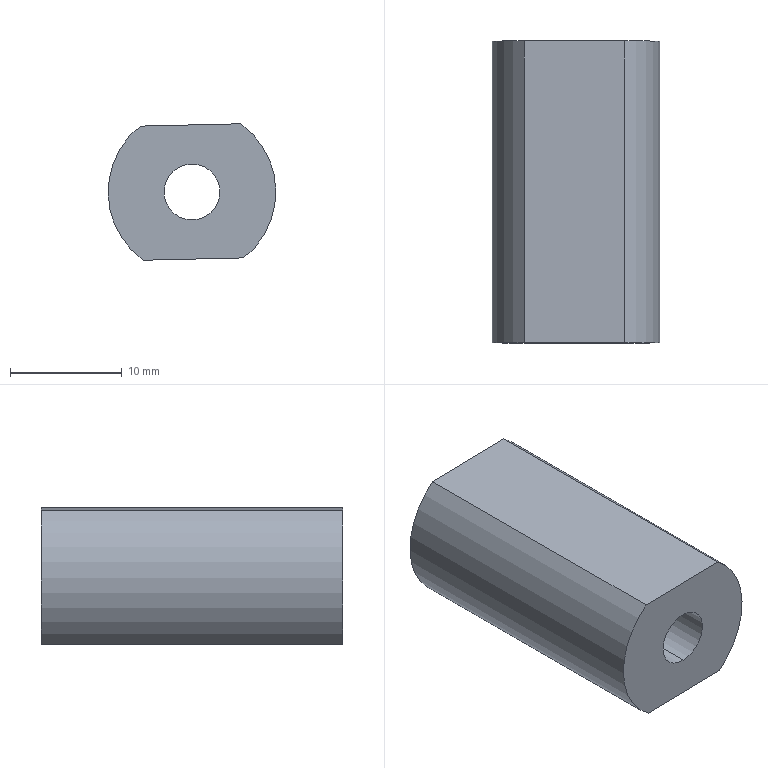Component | SolidWorks | Inline-H010-H01160308-004K-1 | 1 solid | 8 faces | box 15 x 27 x 12.2 mm | volume 3745 mm3 | cylinder 4 | plane 4 | commonest cylinder face diameters 5 x2 15 x2
build123d program:
from build123d import *

# Parameters (mm, degrees)
SKETCH2_W          = 7.5
SKETCH2_H          = 27
SKETCH3_W          = 1.5
SKETCH3_H          = 16
CUT_EXTRUDE1_DEPTH = 15


with BuildPart() as part:
    # Sketch2 → Revolve1 (revolve)
    with BuildSketch(Plane.XY, mode=Mode.PRIVATE) as revolve1_sk:
        with Locations((3.75, 0)):
            Rectangle(SKETCH2_W, SKETCH2_H)
    revolve(revolve1_sk.sketch.rotate(Axis((0, -13.5, 0), (0, 1, 0)), 90), axis=Axis((0, -13.5, 0), (0, 1, 0)))

    # Sketch3 → Cut-Extrude1 (cut, symmetric)
    with BuildSketch(Plane(origin=(0, 0, 0), x_dir=(0, 0, -1), z_dir=(1, 0, 0))):
        with Locations((6.75, -6.484)):
            Rectangle(SKETCH3_W, SKETCH3_H)
        with Locations((-6.75, -6.663)):
            Rectangle(SKETCH3_W, SKETCH3_H)
    cut_extrude1 = extrude(amount=CUT_EXTRUDE1_DEPTH, both=True, mode=Mode.SUBTRACT)

    # Mirror1: Cut-Extrude1 across plane
    add(cut_extrude1.mirror(Plane.ZX), mode=Mode.SUBTRACT)

    # Sketch4 → M6 Tapped Hole1 (revolve, cut)
    with BuildSketch(Plane(origin=(0, 13.5, 0), x_dir=(0, 0, 1), z_dir=(1, 0, 0))):
        Polygon((0, 0), (0, 16.502), (2.5, 15), (2.5, 0), align=None)
    m6_tapped_hole1 = revolve(axis=Axis((0, 19.85, 0), (0, -1, 0)), mode=Mode.SUBTRACT)

    # Mirror2: M6 Tapped Hole1 across plane
    add(m6_tapped_hole1.mirror(Plane.ZX), mode=Mode.SUBTRACT)


solid = part.part

# Placed as in the assembly
solid = solid.moved(Location((-26.521, 7.468, 194.769), (0, -1.316, 180)))
STEP:
#1=COLOUR_RGB('',0.7922,0.8196,0.9333);
#2=FILL_AREA_STYLE_COLOUR('',#1);
#3=FILL_AREA_STYLE('',(#2));
#4=SURFACE_STYLE_FILL_AREA(#3);
#5=SURFACE_SIDE_STYLE('',(#4));
#6=SURFACE_STYLE_USAGE(.BOTH.,#5);
#7=PRESENTATION_STYLE_ASSIGNMENT((#6));
#8=CARTESIAN_POINT('',(-1.046,-0.2375,7.766));
#9=VERTEX_POINT('',#8);
#10=CARTESIAN_POINT('',(-1.042,-0.2375,7.57));
#11=VERTEX_POINT('',#10);
#12=CARTESIAN_POINT('',(-1.044,-0.2375,7.668));
#13=DIRECTION('',(0.,-1.,-0.));
#14=DIRECTION('',(0.02297,0.,-0.9997));
#15=AXIS2_PLACEMENT_3D('',#12,#13,#14);
#16=CIRCLE('',#15,0.09843);
#17=EDGE_CURVE('',#9,#11,#16,.T.);
#18=ORIENTED_EDGE('',*,*,#17,.T.);
#19=CARTESIAN_POINT('',(-1.042,0.8255,7.57));
#20=VERTEX_POINT('',#19);
#21=CARTESIAN_POINT('',(-1.042,0.8255,7.57));
#22=DIRECTION('',(-0.,1.,0.));
#23=VECTOR('',#22,39.37);
#24=LINE('',#21,#23);
#25=EDGE_CURVE('',#11,#20,#24,.T.);
#26=ORIENTED_EDGE('',*,*,#25,.T.);
#27=CARTESIAN_POINT('',(-1.046,0.8255,7.766));
#28=VERTEX_POINT('',#27);
#29=CARTESIAN_POINT('',(-1.044,0.8255,7.668));
#30=DIRECTION('',(-0.,1.,0.));
#31=DIRECTION('',(-0.02297,0.,0.9997));
#32=AXIS2_PLACEMENT_3D('',#29,#30,#31);
#33=CIRCLE('',#32,0.09843);
#34=EDGE_CURVE('',#20,#28,#33,.T.);
#35=ORIENTED_EDGE('',*,*,#34,.T.);
#36=CARTESIAN_POINT('',(-1.046,0.8255,7.766));
#37=DIRECTION('',(-0.,1.,0.));
#38=VECTOR('',#37,39.37);
#39=LINE('',#36,#38);
#40=EDGE_CURVE('',#9,#28,#39,.T.);
#41=ORIENTED_EDGE('',*,*,#40,.F.);
#42=EDGE_LOOP('',(#18,#26,#35,#41));
#43=FACE_OUTER_BOUND('',#42,.T.);
#44=CARTESIAN_POINT('',(-1.044,0.8255,7.668));
#45=DIRECTION('',(-0.,1.,0.));
#46=DIRECTION('',(-0.02297,0.,0.9997));
#47=AXIS2_PLACEMENT_3D('',#44,#45,#46);
#48=CYLINDRICAL_SURFACE('',#47,0.09843);
#49=ADVANCED_FACE('',(#43),#48,.F.);
#50=CARTESIAN_POINT('',(-1.044,0.8255,7.668));
#51=DIRECTION('',(-0.,1.,0.));
#52=DIRECTION('',(-0.02297,0.,0.9997));
#53=AXIS2_PLACEMENT_3D('',#50,#51,#52);
#54=CIRCLE('',#53,0.09843);
#55=EDGE_CURVE('',#28,#20,#54,.T.);
#56=ORIENTED_EDGE('',*,*,#55,.F.);
#57=ORIENTED_EDGE('',*,*,#34,.F.);
#58=EDGE_LOOP('',(#56,#57));
#59=FACE_BOUND('',#58,.T.);
#60=CARTESIAN_POINT('',(-1.227,0.8255,7.9));
#61=VERTEX_POINT('',#60);
#62=CARTESIAN_POINT('',(-1.216,0.8255,7.428));
#63=VERTEX_POINT('',#62);
#64=CARTESIAN_POINT('',(-1.044,0.8255,7.668));
#65=DIRECTION('',(0.,-1.,-0.));
#66=DIRECTION('',(0.02297,0.,-0.9997));
#67=AXIS2_PLACEMENT_3D('',#64,#65,#66);
#68=CIRCLE('',#67,0.2953);
#69=EDGE_CURVE('',#61,#63,#68,.T.);
#70=ORIENTED_EDGE('',*,*,#69,.F.);
#71=CARTESIAN_POINT('',(-0.8724,0.8255,7.908));
#72=VERTEX_POINT('',#71);
#73=CARTESIAN_POINT('',(-1.05,0.8255,7.904));
#74=DIRECTION('',(0.9997,0.,0.02297));
#75=VECTOR('',#74,39.37);
#76=LINE('',#73,#75);
#77=EDGE_CURVE('',#61,#72,#76,.T.);
#78=ORIENTED_EDGE('',*,*,#77,.T.);
#79=CARTESIAN_POINT('',(-0.8616,0.8255,7.436));
#80=VERTEX_POINT('',#79);
#81=CARTESIAN_POINT('',(-1.044,0.8255,7.668));
#82=DIRECTION('',(0.,-1.,-0.));
#83=DIRECTION('',(0.02297,0.,-0.9997));
#84=AXIS2_PLACEMENT_3D('',#81,#82,#83);
#85=CIRCLE('',#84,0.2953);
#86=EDGE_CURVE('',#80,#72,#85,.T.);
#87=ORIENTED_EDGE('',*,*,#86,.F.);
#88=CARTESIAN_POINT('',(-1.039,0.8255,7.432));
#89=DIRECTION('',(-0.9997,-0.,-0.02297));
#90=VECTOR('',#89,39.37);
#91=LINE('',#88,#90);
#92=EDGE_CURVE('',#80,#63,#91,.T.);
#93=ORIENTED_EDGE('',*,*,#92,.T.);
#94=EDGE_LOOP('',(#70,#78,#87,#93));
#95=FACE_OUTER_BOUND('',#94,.T.);
#96=CARTESIAN_POINT('',(-1.044,0.8255,7.668));
#97=DIRECTION('',(-0.,1.,0.));
#98=DIRECTION('',(-0.02297,-0.,0.9997));
#99=AXIS2_PLACEMENT_3D('',#96,#97,#98);
#100=PLANE('',#99);
#101=ADVANCED_FACE('',(#59,#95),#100,.T.);
#102=CARTESIAN_POINT('',(-1.227,-0.2375,7.9));
#103=VERTEX_POINT('',#102);
#104=CARTESIAN_POINT('',(-1.227,-0.2375,7.9));
#105=DIRECTION('',(0.,-1.,-0.));
#106=VECTOR('',#105,39.37);
#107=LINE('',#104,#106);
#108=EDGE_CURVE('',#61,#103,#107,.T.);
#109=ORIENTED_EDGE('',*,*,#108,.F.);
#110=ORIENTED_EDGE('',*,*,#69,.T.);
#111=CARTESIAN_POINT('',(-1.216,-0.2375,7.428));
#112=VERTEX_POINT('',#111);
#113=CARTESIAN_POINT('',(-1.216,-0.2375,7.428));
#114=DIRECTION('',(-0.,1.,0.));
#115=VECTOR('',#114,39.37);
#116=LINE('',#113,#115);
#117=EDGE_CURVE('',#112,#63,#116,.T.);
#118=ORIENTED_EDGE('',*,*,#117,.F.);
#119=CARTESIAN_POINT('',(-1.044,-0.2375,7.668));
#120=DIRECTION('',(0.,-1.,-0.));
#121=DIRECTION('',(0.02297,0.,-0.9997));
#122=AXIS2_PLACEMENT_3D('',#119,#120,#121);
#123=CIRCLE('',#122,0.2953);
#124=EDGE_CURVE('',#103,#112,#123,.T.);
#125=ORIENTED_EDGE('',*,*,#124,.F.);
#126=EDGE_LOOP('',(#109,#110,#118,#125));
#127=FACE_OUTER_BOUND('',#126,.T.);
#128=CARTESIAN_POINT('',(-1.044,-0.2375,7.668));
#129=DIRECTION('',(0.,-1.,-0.));
#130=DIRECTION('',(0.02297,0.,-0.9997));
#131=AXIS2_PLACEMENT_3D('',#128,#129,#130);
#132=CYLINDRICAL_SURFACE('',#131,0.2953);
#133=ADVANCED_FACE('',(#127),#132,.T.);
#134=ORIENTED_EDGE('',*,*,#86,.T.);
#135=CARTESIAN_POINT('',(-0.8724,-0.2375,7.908));
#136=VERTEX_POINT('',#135);
#137=CARTESIAN_POINT('',(-0.8724,-0.2375,7.908));
#138=DIRECTION('',(-0.,1.,0.));
#139=VECTOR('',#138,39.37);
#140=LINE('',#137,#139);
#141=EDGE_CURVE('',#136,#72,#140,.T.);
#142=ORIENTED_EDGE('',*,*,#141,.F.);
#143=CARTESIAN_POINT('',(-0.8616,-0.2375,7.436));
#144=VERTEX_POINT('',#143);
#145=CARTESIAN_POINT('',(-1.044,-0.2375,7.668));
#146=DIRECTION('',(0.,-1.,-0.));
#147=DIRECTION('',(0.02297,0.,-0.9997));
#148=AXIS2_PLACEMENT_3D('',#145,#146,#147);
#149=CIRCLE('',#148,0.2953);
#150=EDGE_CURVE('',#144,#136,#149,.T.);
#151=ORIENTED_EDGE('',*,*,#150,.F.);
#152=CARTESIAN_POINT('',(-0.8616,-0.2375,7.436));
#153=DIRECTION('',(0.,-1.,-0.));
#154=VECTOR('',#153,39.37);
#155=LINE('',#152,#154);
#156=EDGE_CURVE('',#80,#144,#155,.T.);
#157=ORIENTED_EDGE('',*,*,#156,.F.);
#158=EDGE_LOOP('',(#134,#142,#151,#157));
#159=FACE_OUTER_BOUND('',#158,.T.);
#160=CARTESIAN_POINT('',(-1.044,-0.2375,7.668));
#161=DIRECTION('',(0.,-1.,-0.));
#162=DIRECTION('',(0.02297,0.,-0.9997));
#163=AXIS2_PLACEMENT_3D('',#160,#161,#162);
#164=CYLINDRICAL_SURFACE('',#163,0.2953);
#165=ADVANCED_FACE('',(#159),#164,.T.);
#166=ORIENTED_EDGE('',*,*,#17,.F.);
#167=CARTESIAN_POINT('',(-1.044,-0.2375,7.668));
#168=DIRECTION('',(0.,-1.,-0.));
#169=DIRECTION('',(0.02297,0.,-0.9997));
#170=AXIS2_PLACEMENT_3D('',#167,#168,#169);
#171=CIRCLE('',#170,0.09843);
#172=EDGE_CURVE('',#11,#9,#171,.T.);
#173=ORIENTED_EDGE('',*,*,#172,.F.);
#174=EDGE_LOOP('',(#166,#173));
#175=FACE_BOUND('',#174,.T.);
#176=CARTESIAN_POINT('',(-0.7543,-0.2375,7.911));
#177=DIRECTION('',(0.9997,0.,0.02297));
#178=VECTOR('',#177,39.37);
#179=LINE('',#176,#178);
#180=EDGE_CURVE('',#103,#136,#179,.T.);
#181=ORIENTED_EDGE('',*,*,#180,.F.);
#182=ORIENTED_EDGE('',*,*,#124,.T.);
#183=CARTESIAN_POINT('',(-0.7435,-0.2375,7.439));
#184=DIRECTION('',(-0.9997,-0.,-0.02297));
#185=VECTOR('',#184,39.37);
#186=LINE('',#183,#185);
#187=EDGE_CURVE('',#144,#112,#186,.T.);
#188=ORIENTED_EDGE('',*,*,#187,.F.);
#189=ORIENTED_EDGE('',*,*,#150,.T.);
#190=EDGE_LOOP('',(#181,#182,#188,#189));
#191=FACE_OUTER_BOUND('',#190,.T.);
#192=CARTESIAN_POINT('',(-0.7489,-0.2375,7.675));
#193=DIRECTION('',(0.,-1.,-0.));
#194=DIRECTION('',(0.02297,0.,-0.9997));
#195=AXIS2_PLACEMENT_3D('',#192,#193,#194);
#196=PLANE('',#195);
#197=ADVANCED_FACE('',(#175,#191),#196,.T.);
#198=ORIENTED_EDGE('',*,*,#156,.T.);
#199=ORIENTED_EDGE('',*,*,#187,.T.);
#200=ORIENTED_EDGE('',*,*,#117,.T.);
#201=ORIENTED_EDGE('',*,*,#92,.F.);
#202=EDGE_LOOP('',(#198,#199,#200,#201));
#203=FACE_OUTER_BOUND('',#202,.T.);
#204=CARTESIAN_POINT('',(-1.629,0.3537,7.418));
#205=DIRECTION('',(-0.02297,-0.,0.9997));
#206=DIRECTION('',(0.9997,0.,0.02297));
#207=AXIS2_PLACEMENT_3D('',#204,#205,#206);
#208=PLANE('',#207);
#209=ADVANCED_FACE('',(#203),#208,.F.);
#210=ORIENTED_EDGE('',*,*,#108,.T.);
#211=ORIENTED_EDGE('',*,*,#180,.T.);
#212=ORIENTED_EDGE('',*,*,#141,.T.);
#213=ORIENTED_EDGE('',*,*,#77,.F.);
#214=EDGE_LOOP('',(#210,#211,#212,#213));
#215=FACE_OUTER_BOUND('',#214,.T.);
#216=CARTESIAN_POINT('',(-1.64,0.3466,7.891));
#217=DIRECTION('',(0.02297,0.,-0.9997));
#218=DIRECTION('',(-0.9997,-0.,-0.02297));
#219=AXIS2_PLACEMENT_3D('',#216,#217,#218);
#220=PLANE('',#219);
#221=ADVANCED_FACE('',(#215),#220,.F.);
#222=ORIENTED_EDGE('',*,*,#25,.F.);
#223=ORIENTED_EDGE('',*,*,#172,.T.);
#224=ORIENTED_EDGE('',*,*,#40,.T.);
#225=ORIENTED_EDGE('',*,*,#55,.T.);
#226=EDGE_LOOP('',(#222,#223,#224,#225));
#227=FACE_OUTER_BOUND('',#226,.T.);
#228=CARTESIAN_POINT('',(-1.044,0.8255,7.668));
#229=DIRECTION('',(-0.,1.,0.));
#230=DIRECTION('',(-0.02297,0.,0.9997));
#231=AXIS2_PLACEMENT_3D('',#228,#229,#230);
#232=CYLINDRICAL_SURFACE('',#231,0.09843);
#233=ADVANCED_FACE('',(#227),#232,.F.);
#234=CLOSED_SHELL('',(#49,#101,#133,#165,#197,#209,#221,#233));
#235=MANIFOLD_SOLID_BREP('',#234);
#236=STYLED_ITEM('',(#7),#235);
#237=(LENGTH_UNIT()NAMED_UNIT(*)SI_UNIT($,.METRE.));
#238=LENGTH_MEASURE_WITH_UNIT(LENGTH_MEASURE(0.0254),#237);
#239=DIMENSIONAL_EXPONENTS(1.,0.,0.,0.,0.,0.,0.);
#240=(CONVERSION_BASED_UNIT('',#238)LENGTH_UNIT()NAMED_UNIT(#239));
#241=UNCERTAINTY_MEASURE_WITH_UNIT(LENGTH_MEASURE(0.00001),#240,'','');
#242=(NAMED_UNIT(*)PLANE_ANGLE_UNIT()SI_UNIT($,.RADIAN.));
#243=(NAMED_UNIT(*)SI_UNIT($,.STERADIAN.)SOLID_ANGLE_UNIT());
#244=(GEOMETRIC_REPRESENTATION_CONTEXT(3)GLOBAL_UNCERTAINTY_ASSIGNED_CONTEXT((#241))GLOBAL_UNIT_ASSIGNED_CONTEXT((#240,#242,#243))REPRESENTATION_CONTEXT('',''));
#245=MECHANICAL_DESIGN_GEOMETRIC_PRESENTATION_REPRESENTATION('',(#236),#244);
#246=PRESENTATION_LAYER_ASSIGNMENT('','',(#236));
#247=CARTESIAN_POINT('',(0.,0.,0.));
#248=DIRECTION('',(0.,0.,1.));
#249=DIRECTION('',(1.,0.,0.));
#250=AXIS2_PLACEMENT_3D('',#247,#248,#249);
#251=(LENGTH_UNIT()NAMED_UNIT(*)SI_UNIT($,.METRE.));
#252=LENGTH_MEASURE_WITH_UNIT(LENGTH_MEASURE(0.0254),#251);
#253=DIMENSIONAL_EXPONENTS(1.,0.,0.,0.,0.,0.,0.);
#254=(CONVERSION_BASED_UNIT('',#252)LENGTH_UNIT()NAMED_UNIT(#253));
#255=UNCERTAINTY_MEASURE_WITH_UNIT(LENGTH_MEASURE(0.00001),#254,'','');
#256=(NAMED_UNIT(*)PLANE_ANGLE_UNIT()SI_UNIT($,.RADIAN.));
#257=(NAMED_UNIT(*)SI_UNIT($,.STERADIAN.)SOLID_ANGLE_UNIT());
#258=(GEOMETRIC_REPRESENTATION_CONTEXT(3)GLOBAL_UNCERTAINTY_ASSIGNED_CONTEXT((#255))GLOBAL_UNIT_ASSIGNED_CONTEXT((#254,#256,#257))REPRESENTATION_CONTEXT('',''));
#259=ADVANCED_BREP_SHAPE_REPRESENTATION('',(#235,#250),#258);